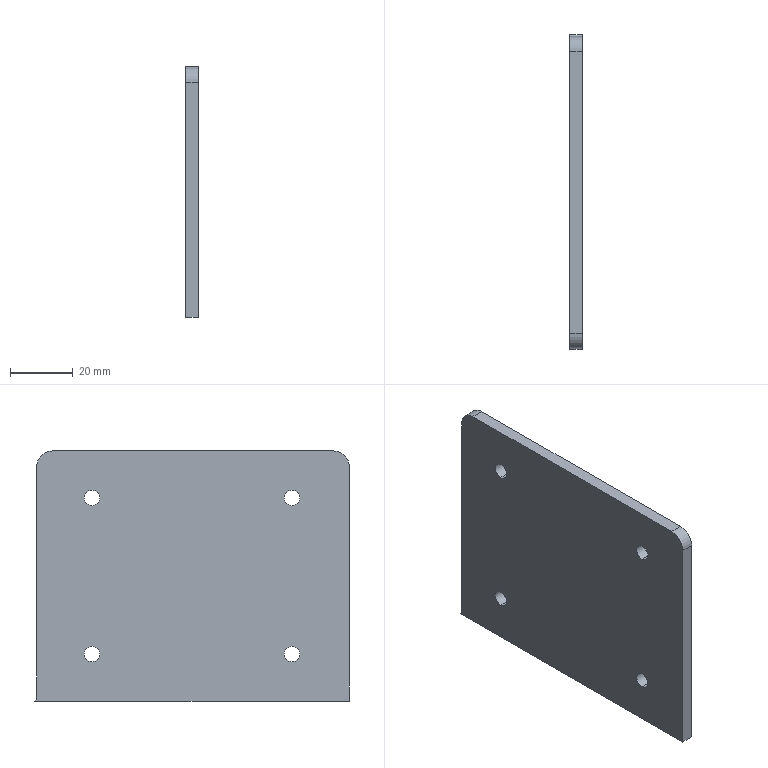Component | SolidWorks | BeltLineSidePlate-1_YL1.sldasm-Part-70-1 | 1 solid | 17 faces | box 4 x 100.63 x 80 mm | volume 31644 mm3 | cylinder 10 | plane 7 | commonest cylinder face diameters 5 x8 10 x2
STEP:
#1=COLOUR_RGB('',0.7922,0.8196,0.9333);
#2=FILL_AREA_STYLE_COLOUR('',#1);
#3=FILL_AREA_STYLE('',(#2));
#4=SURFACE_STYLE_FILL_AREA(#3);
#5=SURFACE_SIDE_STYLE('',(#4));
#6=SURFACE_STYLE_USAGE(.BOTH.,#5);
#7=PRESENTATION_STYLE_ASSIGNMENT((#6));
#8=CARTESIAN_POINT('',(239.961,115.275,2.751));
#9=VERTEX_POINT('',#8);
#10=CARTESIAN_POINT('',(239.961,115.275,2.948));
#11=VERTEX_POINT('',#10);
#12=CARTESIAN_POINT('',(239.961,115.275,2.849));
#13=DIRECTION('',(-1.,-0.,-0.));
#14=DIRECTION('',(0.,0.,1.));
#15=AXIS2_PLACEMENT_3D('',#12,#13,#14);
#16=CIRCLE('',#15,0.09843);
#17=EDGE_CURVE('',#9,#11,#16,.T.);
#18=ORIENTED_EDGE('',*,*,#17,.T.);
#19=CARTESIAN_POINT('',(240.118,115.275,2.948));
#20=VERTEX_POINT('',#19);
#21=CARTESIAN_POINT('',(240.118,115.275,2.948));
#22=DIRECTION('',(1.,0.,0.));
#23=VECTOR('',#22,39.37);
#24=LINE('',#21,#23);
#25=EDGE_CURVE('',#11,#20,#24,.T.);
#26=ORIENTED_EDGE('',*,*,#25,.T.);
#27=CARTESIAN_POINT('',(240.118,115.275,2.751));
#28=VERTEX_POINT('',#27);
#29=CARTESIAN_POINT('',(240.118,115.275,2.849));
#30=DIRECTION('',(1.,0.,0.));
#31=DIRECTION('',(0.,0.,-1.));
#32=AXIS2_PLACEMENT_3D('',#29,#30,#31);
#33=CIRCLE('',#32,0.09843);
#34=EDGE_CURVE('',#20,#28,#33,.T.);
#35=ORIENTED_EDGE('',*,*,#34,.T.);
#36=CARTESIAN_POINT('',(240.118,115.275,2.751));
#37=DIRECTION('',(1.,0.,0.));
#38=VECTOR('',#37,39.37);
#39=LINE('',#36,#38);
#40=EDGE_CURVE('',#9,#28,#39,.T.);
#41=ORIENTED_EDGE('',*,*,#40,.F.);
#42=EDGE_LOOP('',(#18,#26,#35,#41));
#43=FACE_OUTER_BOUND('',#42,.T.);
#44=CARTESIAN_POINT('',(240.118,115.275,2.849));
#45=DIRECTION('',(1.,0.,0.));
#46=DIRECTION('',(0.,0.,-1.));
#47=AXIS2_PLACEMENT_3D('',#44,#45,#46);
#48=CYLINDRICAL_SURFACE('',#47,0.09843);
#49=ADVANCED_FACE('',(#43),#48,.F.);
#50=CARTESIAN_POINT('',(239.961,115.275,0.7825));
#51=VERTEX_POINT('',#50);
#52=CARTESIAN_POINT('',(239.961,115.275,0.9793));
#53=VERTEX_POINT('',#52);
#54=CARTESIAN_POINT('',(239.961,115.275,0.8809));
#55=DIRECTION('',(-1.,-0.,-0.));
#56=DIRECTION('',(0.,0.,1.));
#57=AXIS2_PLACEMENT_3D('',#54,#55,#56);
#58=CIRCLE('',#57,0.09843);
#59=EDGE_CURVE('',#51,#53,#58,.T.);
#60=ORIENTED_EDGE('',*,*,#59,.T.);
#61=CARTESIAN_POINT('',(240.118,115.275,0.9793));
#62=VERTEX_POINT('',#61);
#63=CARTESIAN_POINT('',(240.118,115.275,0.9793));
#64=DIRECTION('',(1.,0.,0.));
#65=VECTOR('',#64,39.37);
#66=LINE('',#63,#65);
#67=EDGE_CURVE('',#53,#62,#66,.T.);
#68=ORIENTED_EDGE('',*,*,#67,.T.);
#69=CARTESIAN_POINT('',(240.118,115.275,0.7825));
#70=VERTEX_POINT('',#69);
#71=CARTESIAN_POINT('',(240.118,115.275,0.8809));
#72=DIRECTION('',(1.,0.,0.));
#73=DIRECTION('',(0.,0.,-1.));
#74=AXIS2_PLACEMENT_3D('',#71,#72,#73);
#75=CIRCLE('',#74,0.09843);
#76=EDGE_CURVE('',#62,#70,#75,.T.);
#77=ORIENTED_EDGE('',*,*,#76,.T.);
#78=CARTESIAN_POINT('',(240.118,115.275,0.7825));
#79=DIRECTION('',(1.,0.,0.));
#80=VECTOR('',#79,39.37);
#81=LINE('',#78,#80);
#82=EDGE_CURVE('',#51,#70,#81,.T.);
#83=ORIENTED_EDGE('',*,*,#82,.F.);
#84=EDGE_LOOP('',(#60,#68,#77,#83));
#85=FACE_OUTER_BOUND('',#84,.T.);
#86=CARTESIAN_POINT('',(240.118,115.275,0.8809));
#87=DIRECTION('',(1.,0.,0.));
#88=DIRECTION('',(0.,0.,-1.));
#89=AXIS2_PLACEMENT_3D('',#86,#87,#88);
#90=CYLINDRICAL_SURFACE('',#89,0.09843);
#91=ADVANCED_FACE('',(#85),#90,.F.);
#92=CARTESIAN_POINT('',(239.961,112.756,2.751));
#93=VERTEX_POINT('',#92);
#94=CARTESIAN_POINT('',(239.961,112.756,2.948));
#95=VERTEX_POINT('',#94);
#96=CARTESIAN_POINT('',(239.961,112.756,2.849));
#97=DIRECTION('',(-1.,-0.,-0.));
#98=DIRECTION('',(0.,0.,1.));
#99=AXIS2_PLACEMENT_3D('',#96,#97,#98);
#100=CIRCLE('',#99,0.09843);
#101=EDGE_CURVE('',#93,#95,#100,.T.);
#102=ORIENTED_EDGE('',*,*,#101,.T.);
#103=CARTESIAN_POINT('',(240.118,112.756,2.948));
#104=VERTEX_POINT('',#103);
#105=CARTESIAN_POINT('',(240.118,112.756,2.948));
#106=DIRECTION('',(1.,0.,0.));
#107=VECTOR('',#106,39.37);
#108=LINE('',#105,#107);
#109=EDGE_CURVE('',#95,#104,#108,.T.);
#110=ORIENTED_EDGE('',*,*,#109,.T.);
#111=CARTESIAN_POINT('',(240.118,112.756,2.751));
#112=VERTEX_POINT('',#111);
#113=CARTESIAN_POINT('',(240.118,112.756,2.849));
#114=DIRECTION('',(1.,0.,0.));
#115=DIRECTION('',(0.,0.,-1.));
#116=AXIS2_PLACEMENT_3D('',#113,#114,#115);
#117=CIRCLE('',#116,0.09843);
#118=EDGE_CURVE('',#104,#112,#117,.T.);
#119=ORIENTED_EDGE('',*,*,#118,.T.);
#120=CARTESIAN_POINT('',(240.118,112.756,2.751));
#121=DIRECTION('',(1.,0.,0.));
#122=VECTOR('',#121,39.37);
#123=LINE('',#120,#122);
#124=EDGE_CURVE('',#93,#112,#123,.T.);
#125=ORIENTED_EDGE('',*,*,#124,.F.);
#126=EDGE_LOOP('',(#102,#110,#119,#125));
#127=FACE_OUTER_BOUND('',#126,.T.);
#128=CARTESIAN_POINT('',(240.118,112.756,2.849));
#129=DIRECTION('',(1.,0.,0.));
#130=DIRECTION('',(0.,0.,-1.));
#131=AXIS2_PLACEMENT_3D('',#128,#129,#130);
#132=CYLINDRICAL_SURFACE('',#131,0.09843);
#133=ADVANCED_FACE('',(#127),#132,.F.);
#134=CARTESIAN_POINT('',(239.961,112.756,0.7825));
#135=VERTEX_POINT('',#134);
#136=CARTESIAN_POINT('',(239.961,112.756,0.9793));
#137=VERTEX_POINT('',#136);
#138=CARTESIAN_POINT('',(239.961,112.756,0.8809));
#139=DIRECTION('',(-1.,-0.,-0.));
#140=DIRECTION('',(0.,0.,1.));
#141=AXIS2_PLACEMENT_3D('',#138,#139,#140);
#142=CIRCLE('',#141,0.09843);
#143=EDGE_CURVE('',#135,#137,#142,.T.);
#144=ORIENTED_EDGE('',*,*,#143,.T.);
#145=CARTESIAN_POINT('',(240.118,112.756,0.9793));
#146=VERTEX_POINT('',#145);
#147=CARTESIAN_POINT('',(240.118,112.756,0.9793));
#148=DIRECTION('',(1.,0.,0.));
#149=VECTOR('',#148,39.37);
#150=LINE('',#147,#149);
#151=EDGE_CURVE('',#137,#146,#150,.T.);
#152=ORIENTED_EDGE('',*,*,#151,.T.);
#153=CARTESIAN_POINT('',(240.118,112.756,0.7825));
#154=VERTEX_POINT('',#153);
#155=CARTESIAN_POINT('',(240.118,112.756,0.8809));
#156=DIRECTION('',(1.,0.,0.));
#157=DIRECTION('',(0.,0.,-1.));
#158=AXIS2_PLACEMENT_3D('',#155,#156,#157);
#159=CIRCLE('',#158,0.09843);
#160=EDGE_CURVE('',#146,#154,#159,.T.);
#161=ORIENTED_EDGE('',*,*,#160,.T.);
#162=CARTESIAN_POINT('',(240.118,112.756,0.7825));
#163=DIRECTION('',(1.,0.,0.));
#164=VECTOR('',#163,39.37);
#165=LINE('',#162,#164);
#166=EDGE_CURVE('',#135,#154,#165,.T.);
#167=ORIENTED_EDGE('',*,*,#166,.F.);
#168=EDGE_LOOP('',(#144,#152,#161,#167));
#169=FACE_OUTER_BOUND('',#168,.T.);
#170=CARTESIAN_POINT('',(240.118,112.756,0.8809));
#171=DIRECTION('',(1.,0.,0.));
#172=DIRECTION('',(0.,0.,-1.));
#173=AXIS2_PLACEMENT_3D('',#170,#171,#172);
#174=CYLINDRICAL_SURFACE('',#173,0.09843);
#175=ADVANCED_FACE('',(#169),#174,.F.);
#176=CARTESIAN_POINT('',(240.118,115.997,0.2904));
#177=VERTEX_POINT('',#176);
#178=CARTESIAN_POINT('',(239.961,115.997,0.2904));
#179=VERTEX_POINT('',#178);
#180=CARTESIAN_POINT('',(240.118,115.997,0.2904));
#181=DIRECTION('',(-1.,-0.,0.));
#182=VECTOR('',#181,39.37);
#183=LINE('',#180,#182);
#184=EDGE_CURVE('',#177,#179,#183,.T.);
#185=ORIENTED_EDGE('',*,*,#184,.F.);
#186=CARTESIAN_POINT('',(240.118,112.035,0.2904));
#187=VERTEX_POINT('',#186);
#188=CARTESIAN_POINT('',(240.118,112.035,0.2904));
#189=DIRECTION('',(0.,-1.,-0.));
#190=VECTOR('',#189,39.37);
#191=LINE('',#188,#190);
#192=EDGE_CURVE('',#177,#187,#191,.T.);
#193=ORIENTED_EDGE('',*,*,#192,.T.);
#194=CARTESIAN_POINT('',(239.961,112.035,0.2904));
#195=VERTEX_POINT('',#194);
#196=CARTESIAN_POINT('',(240.118,112.035,0.2904));
#197=DIRECTION('',(1.,-0.,-0.));
#198=VECTOR('',#197,39.37);
#199=LINE('',#196,#198);
#200=EDGE_CURVE('',#195,#187,#199,.T.);
#201=ORIENTED_EDGE('',*,*,#200,.F.);
#202=CARTESIAN_POINT('',(239.961,112.035,0.2904));
#203=DIRECTION('',(0.,-1.,-0.));
#204=VECTOR('',#203,39.37);
#205=LINE('',#202,#204);
#206=EDGE_CURVE('',#179,#195,#205,.T.);
#207=ORIENTED_EDGE('',*,*,#206,.F.);
#208=EDGE_LOOP('',(#185,#193,#201,#207));
#209=FACE_OUTER_BOUND('',#208,.T.);
#210=CARTESIAN_POINT('',(239.882,114.003,0.2904));
#211=DIRECTION('',(-0.,-0.,-1.));
#212=DIRECTION('',(-1.,-0.,0.));
#213=AXIS2_PLACEMENT_3D('',#210,#211,#212);
#214=PLANE('',#213);
#215=ADVANCED_FACE('',(#209),#214,.T.);
#216=CARTESIAN_POINT('',(240.118,112.035,3.243));
#217=VERTEX_POINT('',#216);
#218=CARTESIAN_POINT('',(240.118,112.035,0.2742));
#219=DIRECTION('',(0.,0.,1.));
#220=VECTOR('',#219,39.37);
#221=LINE('',#218,#220);
#222=EDGE_CURVE('',#187,#217,#221,.T.);
#223=ORIENTED_EDGE('',*,*,#222,.T.);
#224=CARTESIAN_POINT('',(239.961,112.035,3.243));
#225=VERTEX_POINT('',#224);
#226=CARTESIAN_POINT('',(240.118,112.035,3.243));
#227=DIRECTION('',(-1.,-0.,-0.));
#228=VECTOR('',#227,39.37);
#229=LINE('',#226,#228);
#230=EDGE_CURVE('',#217,#225,#229,.T.);
#231=ORIENTED_EDGE('',*,*,#230,.T.);
#232=CARTESIAN_POINT('',(239.961,112.035,0.2742));
#233=DIRECTION('',(0.,0.,1.));
#234=VECTOR('',#233,39.37);
#235=LINE('',#232,#234);
#236=EDGE_CURVE('',#195,#225,#235,.T.);
#237=ORIENTED_EDGE('',*,*,#236,.F.);
#238=ORIENTED_EDGE('',*,*,#200,.T.);
#239=EDGE_LOOP('',(#223,#231,#237,#238));
#240=FACE_OUTER_BOUND('',#239,.T.);
#241=CARTESIAN_POINT('',(240.118,112.035,0.2742));
#242=DIRECTION('',(0.,-1.,0.));
#243=DIRECTION('',(-0.,-0.,-1.));
#244=AXIS2_PLACEMENT_3D('',#241,#242,#243);
#245=PLANE('',#244);
#246=ADVANCED_FACE('',(#240),#245,.T.);
#247=CARTESIAN_POINT('',(240.118,115.972,0.3153));
#248=VERTEX_POINT('',#247);
#249=CARTESIAN_POINT('',(240.118,115.972,0.3153));
#250=DIRECTION('',(-0.,0.7071,-0.7071));
#251=VECTOR('',#250,39.37);
#252=LINE('',#249,#251);
#253=EDGE_CURVE('',#248,#177,#252,.T.);
#254=ORIENTED_EDGE('',*,*,#253,.T.);
#255=ORIENTED_EDGE('',*,*,#184,.T.);
#256=CARTESIAN_POINT('',(239.961,115.972,0.3153));
#257=VERTEX_POINT('',#256);
#258=CARTESIAN_POINT('',(239.961,115.972,0.3153));
#259=DIRECTION('',(-0.,0.7071,-0.7071));
#260=VECTOR('',#259,39.37);
#261=LINE('',#258,#260);
#262=EDGE_CURVE('',#257,#179,#261,.T.);
#263=ORIENTED_EDGE('',*,*,#262,.F.);
#264=CARTESIAN_POINT('',(240.118,115.972,0.3153));
#265=DIRECTION('',(-1.,-0.,-0.));
#266=VECTOR('',#265,39.37);
#267=LINE('',#264,#266);
#268=EDGE_CURVE('',#248,#257,#267,.T.);
#269=ORIENTED_EDGE('',*,*,#268,.F.);
#270=EDGE_LOOP('',(#254,#255,#263,#269));
#271=FACE_OUTER_BOUND('',#270,.T.);
#272=CARTESIAN_POINT('',(240.118,115.972,0.3153));
#273=DIRECTION('',(0.,0.7071,0.7071));
#274=DIRECTION('',(0.,-0.7071,0.7071));
#275=AXIS2_PLACEMENT_3D('',#272,#273,#274);
#276=PLANE('',#275);
#277=ADVANCED_FACE('',(#271),#276,.T.);
#278=CARTESIAN_POINT('',(240.118,115.275,2.849));
#279=DIRECTION('',(1.,0.,0.));
#280=DIRECTION('',(0.,0.,-1.));
#281=AXIS2_PLACEMENT_3D('',#278,#279,#280);
#282=CIRCLE('',#281,0.09843);
#283=EDGE_CURVE('',#28,#20,#282,.T.);
#284=ORIENTED_EDGE('',*,*,#283,.F.);
#285=ORIENTED_EDGE('',*,*,#34,.F.);
#286=EDGE_LOOP('',(#284,#285));
#287=FACE_BOUND('',#286,.T.);
#288=CARTESIAN_POINT('',(240.118,115.275,0.8809));
#289=DIRECTION('',(1.,0.,0.));
#290=DIRECTION('',(0.,0.,-1.));
#291=AXIS2_PLACEMENT_3D('',#288,#289,#290);
#292=CIRCLE('',#291,0.09843);
#293=EDGE_CURVE('',#70,#62,#292,.T.);
#294=ORIENTED_EDGE('',*,*,#293,.F.);
#295=ORIENTED_EDGE('',*,*,#76,.F.);
#296=EDGE_LOOP('',(#294,#295));
#297=FACE_BOUND('',#296,.T.);
#298=CARTESIAN_POINT('',(240.118,112.756,2.849));
#299=DIRECTION('',(1.,0.,0.));
#300=DIRECTION('',(0.,0.,-1.));
#301=AXIS2_PLACEMENT_3D('',#298,#299,#300);
#302=CIRCLE('',#301,0.09843);
#303=EDGE_CURVE('',#112,#104,#302,.T.);
#304=ORIENTED_EDGE('',*,*,#303,.F.);
#305=ORIENTED_EDGE('',*,*,#118,.F.);
#306=EDGE_LOOP('',(#304,#305));
#307=FACE_BOUND('',#306,.T.);
#308=CARTESIAN_POINT('',(240.118,112.756,0.8809));
#309=DIRECTION('',(1.,0.,0.));
#310=DIRECTION('',(0.,0.,-1.));
#311=AXIS2_PLACEMENT_3D('',#308,#309,#310);
#312=CIRCLE('',#311,0.09843);
#313=EDGE_CURVE('',#154,#146,#312,.T.);
#314=ORIENTED_EDGE('',*,*,#313,.F.);
#315=ORIENTED_EDGE('',*,*,#160,.F.);
#316=EDGE_LOOP('',(#314,#315));
#317=FACE_BOUND('',#316,.T.);
#318=CARTESIAN_POINT('',(240.118,115.972,3.243));
#319=VERTEX_POINT('',#318);
#320=CARTESIAN_POINT('',(240.118,115.972,3.44));
#321=DIRECTION('',(-0.,-0.,-1.));
#322=VECTOR('',#321,39.37);
#323=LINE('',#320,#322);
#324=EDGE_CURVE('',#319,#248,#323,.T.);
#325=ORIENTED_EDGE('',*,*,#324,.F.);
#326=CARTESIAN_POINT('',(240.118,115.775,3.44));
#327=VERTEX_POINT('',#326);
#328=CARTESIAN_POINT('',(240.118,115.775,3.243));
#329=DIRECTION('',(1.,0.,0.));
#330=DIRECTION('',(0.,0.,1.));
#331=AXIS2_PLACEMENT_3D('',#328,#329,#330);
#332=CIRCLE('',#331,0.1969);
#333=EDGE_CURVE('',#319,#327,#332,.T.);
#334=ORIENTED_EDGE('',*,*,#333,.T.);
#335=CARTESIAN_POINT('',(240.118,112.231,3.44));
#336=VERTEX_POINT('',#335);
#337=CARTESIAN_POINT('',(240.118,112.035,3.44));
#338=DIRECTION('',(-0.,1.,0.));
#339=VECTOR('',#338,39.37);
#340=LINE('',#337,#339);
#341=EDGE_CURVE('',#336,#327,#340,.T.);
#342=ORIENTED_EDGE('',*,*,#341,.F.);
#343=CARTESIAN_POINT('',(240.118,112.231,3.243));
#344=DIRECTION('',(1.,0.,0.));
#345=DIRECTION('',(0.,0.,1.));
#346=AXIS2_PLACEMENT_3D('',#343,#344,#345);
#347=CIRCLE('',#346,0.1969);
#348=EDGE_CURVE('',#336,#217,#347,.T.);
#349=ORIENTED_EDGE('',*,*,#348,.T.);
#350=ORIENTED_EDGE('',*,*,#222,.F.);
#351=ORIENTED_EDGE('',*,*,#192,.F.);
#352=ORIENTED_EDGE('',*,*,#253,.F.);
#353=EDGE_LOOP('',(#325,#334,#342,#349,#350,#351,#352));
#354=FACE_OUTER_BOUND('',#353,.T.);
#355=CARTESIAN_POINT('',(240.118,112.035,0.2742));
#356=DIRECTION('',(-1.,-0.,0.));
#357=DIRECTION('',(0.,0.,1.));
#358=AXIS2_PLACEMENT_3D('',#355,#356,#357);
#359=PLANE('',#358);
#360=ADVANCED_FACE('',(#287,#297,#307,#317,#354),#359,.F.);
#361=ORIENTED_EDGE('',*,*,#17,.F.);
#362=CARTESIAN_POINT('',(239.961,115.275,2.849));
#363=DIRECTION('',(-1.,-0.,-0.));
#364=DIRECTION('',(0.,0.,1.));
#365=AXIS2_PLACEMENT_3D('',#362,#363,#364);
#366=CIRCLE('',#365,0.09843);
#367=EDGE_CURVE('',#11,#9,#366,.T.);
#368=ORIENTED_EDGE('',*,*,#367,.F.);
#369=EDGE_LOOP('',(#361,#368));
#370=FACE_BOUND('',#369,.T.);
#371=ORIENTED_EDGE('',*,*,#59,.F.);
#372=CARTESIAN_POINT('',(239.961,115.275,0.8809));
#373=DIRECTION('',(-1.,-0.,-0.));
#374=DIRECTION('',(0.,0.,1.));
#375=AXIS2_PLACEMENT_3D('',#372,#373,#374);
#376=CIRCLE('',#375,0.09843);
#377=EDGE_CURVE('',#53,#51,#376,.T.);
#378=ORIENTED_EDGE('',*,*,#377,.F.);
#379=EDGE_LOOP('',(#371,#378));
#380=FACE_BOUND('',#379,.T.);
#381=ORIENTED_EDGE('',*,*,#101,.F.);
#382=CARTESIAN_POINT('',(239.961,112.756,2.849));
#383=DIRECTION('',(-1.,-0.,-0.));
#384=DIRECTION('',(0.,0.,1.));
#385=AXIS2_PLACEMENT_3D('',#382,#383,#384);
#386=CIRCLE('',#385,0.09843);
#387=EDGE_CURVE('',#95,#93,#386,.T.);
#388=ORIENTED_EDGE('',*,*,#387,.F.);
#389=EDGE_LOOP('',(#381,#388));
#390=FACE_BOUND('',#389,.T.);
#391=ORIENTED_EDGE('',*,*,#143,.F.);
#392=CARTESIAN_POINT('',(239.961,112.756,0.8809));
#393=DIRECTION('',(-1.,-0.,-0.));
#394=DIRECTION('',(0.,0.,1.));
#395=AXIS2_PLACEMENT_3D('',#392,#393,#394);
#396=CIRCLE('',#395,0.09843);
#397=EDGE_CURVE('',#137,#135,#396,.T.);
#398=ORIENTED_EDGE('',*,*,#397,.F.);
#399=EDGE_LOOP('',(#391,#398));
#400=FACE_BOUND('',#399,.T.);
#401=CARTESIAN_POINT('',(239.961,112.231,3.44));
#402=VERTEX_POINT('',#401);
#403=CARTESIAN_POINT('',(239.961,115.775,3.44));
#404=VERTEX_POINT('',#403);
#405=CARTESIAN_POINT('',(239.961,112.035,3.44));
#406=DIRECTION('',(-0.,1.,0.));
#407=VECTOR('',#406,39.37);
#408=LINE('',#405,#407);
#409=EDGE_CURVE('',#402,#404,#408,.T.);
#410=ORIENTED_EDGE('',*,*,#409,.T.);
#411=CARTESIAN_POINT('',(239.961,115.972,3.243));
#412=VERTEX_POINT('',#411);
#413=CARTESIAN_POINT('',(239.961,115.775,3.243));
#414=DIRECTION('',(-1.,-0.,-0.));
#415=DIRECTION('',(0.,0.,1.));
#416=AXIS2_PLACEMENT_3D('',#413,#414,#415);
#417=CIRCLE('',#416,0.1969);
#418=EDGE_CURVE('',#404,#412,#417,.T.);
#419=ORIENTED_EDGE('',*,*,#418,.T.);
#420=CARTESIAN_POINT('',(239.961,115.972,3.44));
#421=DIRECTION('',(-0.,-0.,-1.));
#422=VECTOR('',#421,39.37);
#423=LINE('',#420,#422);
#424=EDGE_CURVE('',#412,#257,#423,.T.);
#425=ORIENTED_EDGE('',*,*,#424,.T.);
#426=ORIENTED_EDGE('',*,*,#262,.T.);
#427=ORIENTED_EDGE('',*,*,#206,.T.);
#428=ORIENTED_EDGE('',*,*,#236,.T.);
#429=CARTESIAN_POINT('',(239.961,112.231,3.243));
#430=DIRECTION('',(-1.,-0.,-0.));
#431=DIRECTION('',(0.,0.,1.));
#432=AXIS2_PLACEMENT_3D('',#429,#430,#431);
#433=CIRCLE('',#432,0.1969);
#434=EDGE_CURVE('',#225,#402,#433,.T.);
#435=ORIENTED_EDGE('',*,*,#434,.T.);
#436=EDGE_LOOP('',(#410,#419,#425,#426,#427,#428,#435));
#437=FACE_OUTER_BOUND('',#436,.T.);
#438=CARTESIAN_POINT('',(239.961,112.035,0.2742));
#439=DIRECTION('',(-1.,-0.,0.));
#440=DIRECTION('',(0.,0.,1.));
#441=AXIS2_PLACEMENT_3D('',#438,#439,#440);
#442=PLANE('',#441);
#443=ADVANCED_FACE('',(#370,#380,#390,#400,#437),#442,.T.);
#444=ORIENTED_EDGE('',*,*,#341,.T.);
#445=CARTESIAN_POINT('',(240.118,115.775,3.44));
#446=DIRECTION('',(-1.,-0.,-0.));
#447=VECTOR('',#446,39.37);
#448=LINE('',#445,#447);
#449=EDGE_CURVE('',#327,#404,#448,.T.);
#450=ORIENTED_EDGE('',*,*,#449,.T.);
#451=ORIENTED_EDGE('',*,*,#409,.F.);
#452=CARTESIAN_POINT('',(240.118,112.231,3.44));
#453=DIRECTION('',(1.,0.,0.));
#454=VECTOR('',#453,39.37);
#455=LINE('',#452,#454);
#456=EDGE_CURVE('',#402,#336,#455,.T.);
#457=ORIENTED_EDGE('',*,*,#456,.T.);
#458=EDGE_LOOP('',(#444,#450,#451,#457));
#459=FACE_OUTER_BOUND('',#458,.T.);
#460=CARTESIAN_POINT('',(240.118,112.035,3.44));
#461=DIRECTION('',(-0.,0.,1.));
#462=DIRECTION('',(1.,0.,0.));
#463=AXIS2_PLACEMENT_3D('',#460,#461,#462);
#464=PLANE('',#463);
#465=ADVANCED_FACE('',(#459),#464,.T.);
#466=ORIENTED_EDGE('',*,*,#424,.F.);
#467=CARTESIAN_POINT('',(240.118,115.972,3.243));
#468=DIRECTION('',(1.,0.,0.));
#469=VECTOR('',#468,39.37);
#470=LINE('',#467,#469);
#471=EDGE_CURVE('',#412,#319,#470,.T.);
#472=ORIENTED_EDGE('',*,*,#471,.T.);
#473=ORIENTED_EDGE('',*,*,#324,.T.);
#474=ORIENTED_EDGE('',*,*,#268,.T.);
#475=EDGE_LOOP('',(#466,#472,#473,#474));
#476=FACE_OUTER_BOUND('',#475,.T.);
#477=CARTESIAN_POINT('',(240.118,115.972,3.44));
#478=DIRECTION('',(-0.,1.,-0.));
#479=DIRECTION('',(0.,0.,1.));
#480=AXIS2_PLACEMENT_3D('',#477,#478,#479);
#481=PLANE('',#480);
#482=ADVANCED_FACE('',(#476),#481,.T.);
#483=ORIENTED_EDGE('',*,*,#333,.F.);
#484=ORIENTED_EDGE('',*,*,#471,.F.);
#485=ORIENTED_EDGE('',*,*,#418,.F.);
#486=ORIENTED_EDGE('',*,*,#449,.F.);
#487=EDGE_LOOP('',(#483,#484,#485,#486));
#488=FACE_OUTER_BOUND('',#487,.T.);
#489=CARTESIAN_POINT('',(240.118,115.775,3.243));
#490=DIRECTION('',(-1.,-0.,-0.));
#491=DIRECTION('',(0.,0.,1.));
#492=AXIS2_PLACEMENT_3D('',#489,#490,#491);
#493=CYLINDRICAL_SURFACE('',#492,0.1969);
#494=ADVANCED_FACE('',(#488),#493,.T.);
#495=ORIENTED_EDGE('',*,*,#348,.F.);
#496=ORIENTED_EDGE('',*,*,#456,.F.);
#497=ORIENTED_EDGE('',*,*,#434,.F.);
#498=ORIENTED_EDGE('',*,*,#230,.F.);
#499=EDGE_LOOP('',(#495,#496,#497,#498));
#500=FACE_OUTER_BOUND('',#499,.T.);
#501=CARTESIAN_POINT('',(240.118,112.231,3.243));
#502=DIRECTION('',(-1.,-0.,-0.));
#503=DIRECTION('',(0.,0.,1.));
#504=AXIS2_PLACEMENT_3D('',#501,#502,#503);
#505=CYLINDRICAL_SURFACE('',#504,0.1969);
#506=ADVANCED_FACE('',(#500),#505,.T.);
#507=ORIENTED_EDGE('',*,*,#151,.F.);
#508=ORIENTED_EDGE('',*,*,#397,.T.);
#509=ORIENTED_EDGE('',*,*,#166,.T.);
#510=ORIENTED_EDGE('',*,*,#313,.T.);
#511=EDGE_LOOP('',(#507,#508,#509,#510));
#512=FACE_OUTER_BOUND('',#511,.T.);
#513=CARTESIAN_POINT('',(240.118,112.756,0.8809));
#514=DIRECTION('',(1.,0.,0.));
#515=DIRECTION('',(0.,0.,-1.));
#516=AXIS2_PLACEMENT_3D('',#513,#514,#515);
#517=CYLINDRICAL_SURFACE('',#516,0.09843);
#518=ADVANCED_FACE('',(#512),#517,.F.);
#519=ORIENTED_EDGE('',*,*,#109,.F.);
#520=ORIENTED_EDGE('',*,*,#387,.T.);
#521=ORIENTED_EDGE('',*,*,#124,.T.);
#522=ORIENTED_EDGE('',*,*,#303,.T.);
#523=EDGE_LOOP('',(#519,#520,#521,#522));
#524=FACE_OUTER_BOUND('',#523,.T.);
#525=CARTESIAN_POINT('',(240.118,112.756,2.849));
#526=DIRECTION('',(1.,0.,0.));
#527=DIRECTION('',(0.,0.,-1.));
#528=AXIS2_PLACEMENT_3D('',#525,#526,#527);
#529=CYLINDRICAL_SURFACE('',#528,0.09843);
#530=ADVANCED_FACE('',(#524),#529,.F.);
#531=ORIENTED_EDGE('',*,*,#67,.F.);
#532=ORIENTED_EDGE('',*,*,#377,.T.);
#533=ORIENTED_EDGE('',*,*,#82,.T.);
#534=ORIENTED_EDGE('',*,*,#293,.T.);
#535=EDGE_LOOP('',(#531,#532,#533,#534));
#536=FACE_OUTER_BOUND('',#535,.T.);
#537=CARTESIAN_POINT('',(240.118,115.275,0.8809));
#538=DIRECTION('',(1.,0.,0.));
#539=DIRECTION('',(0.,0.,-1.));
#540=AXIS2_PLACEMENT_3D('',#537,#538,#539);
#541=CYLINDRICAL_SURFACE('',#540,0.09843);
#542=ADVANCED_FACE('',(#536),#541,.F.);
#543=ORIENTED_EDGE('',*,*,#25,.F.);
#544=ORIENTED_EDGE('',*,*,#367,.T.);
#545=ORIENTED_EDGE('',*,*,#40,.T.);
#546=ORIENTED_EDGE('',*,*,#283,.T.);
#547=EDGE_LOOP('',(#543,#544,#545,#546));
#548=FACE_OUTER_BOUND('',#547,.T.);
#549=CARTESIAN_POINT('',(240.118,115.275,2.849));
#550=DIRECTION('',(1.,0.,0.));
#551=DIRECTION('',(0.,0.,-1.));
#552=AXIS2_PLACEMENT_3D('',#549,#550,#551);
#553=CYLINDRICAL_SURFACE('',#552,0.09843);
#554=ADVANCED_FACE('',(#548),#553,.F.);
#555=CLOSED_SHELL('',(#49,#91,#133,#175,#215,#246,#277,#360,#443,#465,#482,#494,#506,#518,#530,#542,#554));
#556=MANIFOLD_SOLID_BREP('',#555);
#557=STYLED_ITEM('',(#7),#556);
#558=PRESENTATION_LAYER_ASSIGNMENT('','',(#557));
#559=(LENGTH_UNIT()NAMED_UNIT(*)SI_UNIT($,.METRE.));
#560=LENGTH_MEASURE_WITH_UNIT(LENGTH_MEASURE(0.0254),#559);
#561=DIMENSIONAL_EXPONENTS(1.,0.,0.,0.,0.,0.,0.);
#562=(CONVERSION_BASED_UNIT('',#560)LENGTH_UNIT()NAMED_UNIT(#561));
#563=UNCERTAINTY_MEASURE_WITH_UNIT(LENGTH_MEASURE(0.00001),#562,'','');
#564=(NAMED_UNIT(*)PLANE_ANGLE_UNIT()SI_UNIT($,.RADIAN.));
#565=(NAMED_UNIT(*)SI_UNIT($,.STERADIAN.)SOLID_ANGLE_UNIT());
#566=(GEOMETRIC_REPRESENTATION_CONTEXT(3)GLOBAL_UNCERTAINTY_ASSIGNED_CONTEXT((#563))GLOBAL_UNIT_ASSIGNED_CONTEXT((#562,#564,#565))REPRESENTATION_CONTEXT('',''));
#567=MECHANICAL_DESIGN_GEOMETRIC_PRESENTATION_REPRESENTATION('',(#557),#566);
#568=CARTESIAN_POINT('',(0.,0.,0.));
#569=DIRECTION('',(0.,0.,1.));
#570=DIRECTION('',(1.,0.,0.));
#571=AXIS2_PLACEMENT_3D('',#568,#569,#570);
#572=(LENGTH_UNIT()NAMED_UNIT(*)SI_UNIT($,.METRE.));
#573=LENGTH_MEASURE_WITH_UNIT(LENGTH_MEASURE(0.0254),#572);
#574=DIMENSIONAL_EXPONENTS(1.,0.,0.,0.,0.,0.,0.);
#575=(CONVERSION_BASED_UNIT('',#573)LENGTH_UNIT()NAMED_UNIT(#574));
#576=UNCERTAINTY_MEASURE_WITH_UNIT(LENGTH_MEASURE(0.00001),#575,'','');
#577=(NAMED_UNIT(*)PLANE_ANGLE_UNIT()SI_UNIT($,.RADIAN.));
#578=(NAMED_UNIT(*)SI_UNIT($,.STERADIAN.)SOLID_ANGLE_UNIT());
#579=(GEOMETRIC_REPRESENTATION_CONTEXT(3)GLOBAL_UNCERTAINTY_ASSIGNED_CONTEXT((#576))GLOBAL_UNIT_ASSIGNED_CONTEXT((#575,#577,#578))REPRESENTATION_CONTEXT('',''));
#580=ADVANCED_BREP_SHAPE_REPRESENTATION('',(#556,#571),#579);